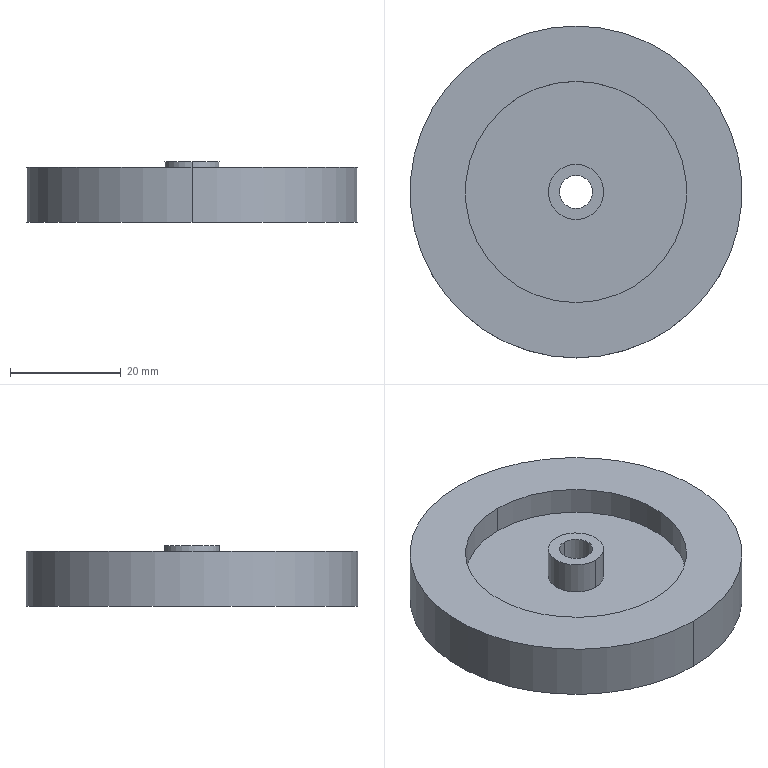Component | SolidWorks | DriveStripPlate-1 | 1 solid | 12 faces | box 60 x 60 x 11 mm | volume 22151 mm3 | cylinder 8 | plane 4 | commonest cylinder face diameters 10 x2 6 x2 60 x2 40 x2
build123d program:
from build123d import *

# Parameters (mm, degrees)
SKETCH1_R           = 30
SKETCH1_R_2         = 20
BOSS_EXTRUDE1_DEPTH = 10
SKETCH2_R           = 20
SKETCH2_R_2         = 3
BOSS_EXTRUDE2_DEPTH = 5
SKETCH3_R           = 5
SKETCH3_R_2         = 3
BOSS_EXTRUDE3_DEPTH = 6


with BuildPart() as part:
    # Sketch1 → Boss-Extrude1 (new body)
    with BuildSketch(Plane.XY):
        with Locations((71.434, 305)):
            Circle(SKETCH1_R)
        with Locations((71.434, 305)):
            Circle(SKETCH1_R_2, mode=Mode.SUBTRACT)
    extrude(amount=BOSS_EXTRUDE1_DEPTH)

    # Sketch2 → Boss-Extrude2 (add)
    with BuildSketch(Plane(origin=(0, 0, 0), x_dir=(-1, 0, 0), z_dir=(0, 0, -1))):
        with Locations((-71.434, 305)):
            Circle(SKETCH2_R)
        with Locations((-71.434, 305)):
            Circle(SKETCH2_R_2, mode=Mode.SUBTRACT)
    extrude(amount=-BOSS_EXTRUDE2_DEPTH)

    # Sketch3 → Boss-Extrude3 (add)
    with BuildSketch(Plane.XY.offset(5)):
        with Locations(Location((71.434, 305, 0), (0, 0, 180))):
            Circle(SKETCH3_R)
        with Locations(Location((71.434, 305, 0), (0, 0, 180))):
            Circle(SKETCH3_R_2, mode=Mode.SUBTRACT)
    extrude(amount=BOSS_EXTRUDE3_DEPTH)


solid = part.part

# Placed as in the assembly
solid = solid.moved(Location((-511.434, -213, 50), (0, 0, 0)))
STEP:
#1=CARTESIAN_POINT('',(-17.323,3.819,2.402));
#2=VERTEX_POINT('',#1);
#3=CARTESIAN_POINT('',(-17.323,3.425,2.402));
#4=VERTEX_POINT('',#3);
#5=CARTESIAN_POINT('',(-17.323,3.622,2.402));
#6=DIRECTION('',(0.,0.,1.));
#7=DIRECTION('',(0.,1.,0.));
#8=AXIS2_PLACEMENT_3D('',#5,#6,#7);
#9=CIRCLE('',#8,0.1969);
#10=EDGE_CURVE('',#2,#4,#9,.T.);
#11=ORIENTED_EDGE('',*,*,#10,.F.);
#12=CARTESIAN_POINT('',(-17.323,3.819,2.165));
#13=VERTEX_POINT('',#12);
#14=CARTESIAN_POINT('',(-17.323,3.819,2.402));
#15=DIRECTION('',(0.,0.,-1.));
#16=VECTOR('',#15,39.37);
#17=LINE('',#14,#16);
#18=EDGE_CURVE('',#2,#13,#17,.T.);
#19=ORIENTED_EDGE('',*,*,#18,.T.);
#20=CARTESIAN_POINT('',(-17.323,3.425,2.165));
#21=VERTEX_POINT('',#20);
#22=CARTESIAN_POINT('',(-17.323,3.622,2.165));
#23=DIRECTION('',(0.,0.,1.));
#24=DIRECTION('',(0.,-1.,0.));
#25=AXIS2_PLACEMENT_3D('',#22,#23,#24);
#26=CIRCLE('',#25,0.1969);
#27=EDGE_CURVE('',#13,#21,#26,.T.);
#28=ORIENTED_EDGE('',*,*,#27,.T.);
#29=CARTESIAN_POINT('',(-17.323,3.425,2.402));
#30=DIRECTION('',(0.,0.,-1.));
#31=VECTOR('',#30,39.37);
#32=LINE('',#29,#31);
#33=EDGE_CURVE('',#4,#21,#32,.T.);
#34=ORIENTED_EDGE('',*,*,#33,.F.);
#35=EDGE_LOOP('',(#11,#19,#28,#34));
#36=FACE_OUTER_BOUND('',#35,.T.);
#37=CARTESIAN_POINT('',(-17.323,3.622,2.402));
#38=DIRECTION('',(0.,0.,-1.));
#39=DIRECTION('',(0.,-1.,0.));
#40=AXIS2_PLACEMENT_3D('',#37,#38,#39);
#41=CYLINDRICAL_SURFACE('',#40,0.1969);
#42=ADVANCED_FACE('',(#36),#41,.T.);
#43=CARTESIAN_POINT('',(-17.323,3.504,2.402));
#44=VERTEX_POINT('',#43);
#45=CARTESIAN_POINT('',(-17.323,3.74,2.402));
#46=VERTEX_POINT('',#45);
#47=CARTESIAN_POINT('',(-17.323,3.622,2.402));
#48=DIRECTION('',(0.,0.,1.));
#49=DIRECTION('',(0.,1.,0.));
#50=AXIS2_PLACEMENT_3D('',#47,#48,#49);
#51=CIRCLE('',#50,0.1181);
#52=EDGE_CURVE('',#44,#46,#51,.T.);
#53=ORIENTED_EDGE('',*,*,#52,.T.);
#54=CARTESIAN_POINT('',(-17.323,3.74,1.969));
#55=VERTEX_POINT('',#54);
#56=CARTESIAN_POINT('',(-17.323,3.74,2.165));
#57=DIRECTION('',(0.,0.,-1.));
#58=VECTOR('',#57,39.37);
#59=LINE('',#56,#58);
#60=EDGE_CURVE('',#46,#55,#59,.T.);
#61=ORIENTED_EDGE('',*,*,#60,.T.);
#62=CARTESIAN_POINT('',(-17.323,3.504,1.969));
#63=VERTEX_POINT('',#62);
#64=CARTESIAN_POINT('',(-17.323,3.622,1.969));
#65=DIRECTION('',(0.,0.,-1.));
#66=DIRECTION('',(0.,-1.,0.));
#67=AXIS2_PLACEMENT_3D('',#64,#65,#66);
#68=CIRCLE('',#67,0.1181);
#69=EDGE_CURVE('',#55,#63,#68,.T.);
#70=ORIENTED_EDGE('',*,*,#69,.T.);
#71=CARTESIAN_POINT('',(-17.323,3.504,2.165));
#72=DIRECTION('',(0.,0.,-1.));
#73=VECTOR('',#72,39.37);
#74=LINE('',#71,#73);
#75=EDGE_CURVE('',#44,#63,#74,.T.);
#76=ORIENTED_EDGE('',*,*,#75,.F.);
#77=EDGE_LOOP('',(#53,#61,#70,#76));
#78=FACE_OUTER_BOUND('',#77,.T.);
#79=CARTESIAN_POINT('',(-17.323,3.622,2.165));
#80=DIRECTION('',(0.,0.,-1.));
#81=DIRECTION('',(0.,-1.,0.));
#82=AXIS2_PLACEMENT_3D('',#79,#80,#81);
#83=CYLINDRICAL_SURFACE('',#82,0.1181);
#84=ADVANCED_FACE('',(#78),#83,.F.);
#85=CARTESIAN_POINT('',(-17.323,4.803,2.362));
#86=VERTEX_POINT('',#85);
#87=CARTESIAN_POINT('',(-17.323,2.441,2.362));
#88=VERTEX_POINT('',#87);
#89=CARTESIAN_POINT('',(-17.323,3.622,2.362));
#90=DIRECTION('',(0.,0.,1.));
#91=DIRECTION('',(0.,1.,0.));
#92=AXIS2_PLACEMENT_3D('',#89,#90,#91);
#93=CIRCLE('',#92,1.181);
#94=EDGE_CURVE('',#86,#88,#93,.T.);
#95=ORIENTED_EDGE('',*,*,#94,.F.);
#96=CARTESIAN_POINT('',(-17.323,4.803,1.969));
#97=VERTEX_POINT('',#96);
#98=CARTESIAN_POINT('',(-17.323,4.803,2.362));
#99=DIRECTION('',(0.,0.,-1.));
#100=VECTOR('',#99,39.37);
#101=LINE('',#98,#100);
#102=EDGE_CURVE('',#86,#97,#101,.T.);
#103=ORIENTED_EDGE('',*,*,#102,.T.);
#104=CARTESIAN_POINT('',(-17.323,2.441,1.969));
#105=VERTEX_POINT('',#104);
#106=CARTESIAN_POINT('',(-17.323,3.622,1.969));
#107=DIRECTION('',(0.,0.,1.));
#108=DIRECTION('',(0.,1.,0.));
#109=AXIS2_PLACEMENT_3D('',#106,#107,#108);
#110=CIRCLE('',#109,1.181);
#111=EDGE_CURVE('',#97,#105,#110,.T.);
#112=ORIENTED_EDGE('',*,*,#111,.T.);
#113=CARTESIAN_POINT('',(-17.323,2.441,2.362));
#114=DIRECTION('',(0.,0.,-1.));
#115=VECTOR('',#114,39.37);
#116=LINE('',#113,#115);
#117=EDGE_CURVE('',#88,#105,#116,.T.);
#118=ORIENTED_EDGE('',*,*,#117,.F.);
#119=EDGE_LOOP('',(#95,#103,#112,#118));
#120=FACE_OUTER_BOUND('',#119,.T.);
#121=CARTESIAN_POINT('',(-17.323,3.622,2.362));
#122=DIRECTION('',(0.,0.,-1.));
#123=DIRECTION('',(0.,-1.,0.));
#124=AXIS2_PLACEMENT_3D('',#121,#122,#123);
#125=CYLINDRICAL_SURFACE('',#124,1.181);
#126=ADVANCED_FACE('',(#120),#125,.T.);
#127=CARTESIAN_POINT('',(-17.323,2.835,2.362));
#128=VERTEX_POINT('',#127);
#129=CARTESIAN_POINT('',(-17.323,4.409,2.362));
#130=VERTEX_POINT('',#129);
#131=CARTESIAN_POINT('',(-17.323,3.622,2.362));
#132=DIRECTION('',(0.,0.,1.));
#133=DIRECTION('',(0.,1.,0.));
#134=AXIS2_PLACEMENT_3D('',#131,#132,#133);
#135=CIRCLE('',#134,0.7874);
#136=EDGE_CURVE('',#128,#130,#135,.T.);
#137=ORIENTED_EDGE('',*,*,#136,.T.);
#138=CARTESIAN_POINT('',(-17.323,4.409,2.165));
#139=VERTEX_POINT('',#138);
#140=CARTESIAN_POINT('',(-17.323,4.409,2.362));
#141=DIRECTION('',(0.,0.,-1.));
#142=VECTOR('',#141,39.37);
#143=LINE('',#140,#142);
#144=EDGE_CURVE('',#130,#139,#143,.T.);
#145=ORIENTED_EDGE('',*,*,#144,.T.);
#146=CARTESIAN_POINT('',(-17.323,2.835,2.165));
#147=VERTEX_POINT('',#146);
#148=CARTESIAN_POINT('',(-17.323,3.622,2.165));
#149=DIRECTION('',(0.,0.,-1.));
#150=DIRECTION('',(0.,-1.,0.));
#151=AXIS2_PLACEMENT_3D('',#148,#149,#150);
#152=CIRCLE('',#151,0.7874);
#153=EDGE_CURVE('',#139,#147,#152,.T.);
#154=ORIENTED_EDGE('',*,*,#153,.T.);
#155=CARTESIAN_POINT('',(-17.323,2.835,2.362));
#156=DIRECTION('',(0.,0.,-1.));
#157=VECTOR('',#156,39.37);
#158=LINE('',#155,#157);
#159=EDGE_CURVE('',#128,#147,#158,.T.);
#160=ORIENTED_EDGE('',*,*,#159,.F.);
#161=EDGE_LOOP('',(#137,#145,#154,#160));
#162=FACE_OUTER_BOUND('',#161,.T.);
#163=CARTESIAN_POINT('',(-17.323,3.622,2.362));
#164=DIRECTION('',(0.,0.,-1.));
#165=DIRECTION('',(0.,-1.,0.));
#166=AXIS2_PLACEMENT_3D('',#163,#164,#165);
#167=CYLINDRICAL_SURFACE('',#166,0.7874);
#168=ADVANCED_FACE('',(#162),#167,.F.);
#169=CARTESIAN_POINT('',(-17.323,3.622,2.165));
#170=DIRECTION('',(0.,0.,-1.));
#171=DIRECTION('',(0.,-1.,0.));
#172=AXIS2_PLACEMENT_3D('',#169,#170,#171);
#173=CIRCLE('',#172,0.7874);
#174=EDGE_CURVE('',#147,#139,#173,.T.);
#175=ORIENTED_EDGE('',*,*,#174,.F.);
#176=ORIENTED_EDGE('',*,*,#153,.F.);
#177=EDGE_LOOP('',(#175,#176));
#178=FACE_OUTER_BOUND('',#177,.T.);
#179=CARTESIAN_POINT('',(-17.323,3.622,2.165));
#180=DIRECTION('',(0.,0.,1.));
#181=DIRECTION('',(0.,-1.,0.));
#182=AXIS2_PLACEMENT_3D('',#179,#180,#181);
#183=CIRCLE('',#182,0.1969);
#184=EDGE_CURVE('',#21,#13,#183,.T.);
#185=ORIENTED_EDGE('',*,*,#184,.F.);
#186=ORIENTED_EDGE('',*,*,#27,.F.);
#187=EDGE_LOOP('',(#185,#186));
#188=FACE_BOUND('',#187,.T.);
#189=CARTESIAN_POINT('',(-17.323,3.622,2.165));
#190=DIRECTION('',(0.,0.,-1.));
#191=DIRECTION('',(0.,-1.,0.));
#192=AXIS2_PLACEMENT_3D('',#189,#190,#191);
#193=PLANE('',#192);
#194=ADVANCED_FACE('',(#178,#188),#193,.F.);
#195=ORIENTED_EDGE('',*,*,#144,.F.);
#196=CARTESIAN_POINT('',(-17.323,3.622,2.362));
#197=DIRECTION('',(0.,0.,1.));
#198=DIRECTION('',(0.,1.,0.));
#199=AXIS2_PLACEMENT_3D('',#196,#197,#198);
#200=CIRCLE('',#199,0.7874);
#201=EDGE_CURVE('',#130,#128,#200,.T.);
#202=ORIENTED_EDGE('',*,*,#201,.T.);
#203=ORIENTED_EDGE('',*,*,#159,.T.);
#204=ORIENTED_EDGE('',*,*,#174,.T.);
#205=EDGE_LOOP('',(#195,#202,#203,#204));
#206=FACE_OUTER_BOUND('',#205,.T.);
#207=CARTESIAN_POINT('',(-17.323,3.622,2.362));
#208=DIRECTION('',(0.,0.,-1.));
#209=DIRECTION('',(0.,-1.,0.));
#210=AXIS2_PLACEMENT_3D('',#207,#208,#209);
#211=CYLINDRICAL_SURFACE('',#210,0.7874);
#212=ADVANCED_FACE('',(#206),#211,.F.);
#213=CARTESIAN_POINT('',(-17.323,3.622,2.362));
#214=DIRECTION('',(0.,0.,1.));
#215=DIRECTION('',(0.,1.,0.));
#216=AXIS2_PLACEMENT_3D('',#213,#214,#215);
#217=CIRCLE('',#216,1.181);
#218=EDGE_CURVE('',#88,#86,#217,.T.);
#219=ORIENTED_EDGE('',*,*,#218,.T.);
#220=ORIENTED_EDGE('',*,*,#94,.T.);
#221=EDGE_LOOP('',(#219,#220));
#222=FACE_OUTER_BOUND('',#221,.T.);
#223=ORIENTED_EDGE('',*,*,#136,.F.);
#224=ORIENTED_EDGE('',*,*,#201,.F.);
#225=EDGE_LOOP('',(#223,#224));
#226=FACE_BOUND('',#225,.T.);
#227=CARTESIAN_POINT('',(-17.323,3.622,2.362));
#228=DIRECTION('',(0.,0.,1.));
#229=DIRECTION('',(0.,1.,0.));
#230=AXIS2_PLACEMENT_3D('',#227,#228,#229);
#231=PLANE('',#230);
#232=ADVANCED_FACE('',(#222,#226),#231,.T.);
#233=CARTESIAN_POINT('',(-17.323,3.622,1.969));
#234=DIRECTION('',(0.,0.,1.));
#235=DIRECTION('',(0.,1.,0.));
#236=AXIS2_PLACEMENT_3D('',#233,#234,#235);
#237=CIRCLE('',#236,1.181);
#238=EDGE_CURVE('',#105,#97,#237,.T.);
#239=ORIENTED_EDGE('',*,*,#238,.F.);
#240=ORIENTED_EDGE('',*,*,#111,.F.);
#241=EDGE_LOOP('',(#239,#240));
#242=FACE_OUTER_BOUND('',#241,.T.);
#243=CARTESIAN_POINT('',(-17.323,3.622,1.969));
#244=DIRECTION('',(0.,0.,-1.));
#245=DIRECTION('',(0.,-1.,0.));
#246=AXIS2_PLACEMENT_3D('',#243,#244,#245);
#247=CIRCLE('',#246,0.1181);
#248=EDGE_CURVE('',#63,#55,#247,.T.);
#249=ORIENTED_EDGE('',*,*,#248,.F.);
#250=ORIENTED_EDGE('',*,*,#69,.F.);
#251=EDGE_LOOP('',(#249,#250));
#252=FACE_BOUND('',#251,.T.);
#253=CARTESIAN_POINT('',(-17.323,3.622,1.969));
#254=DIRECTION('',(0.,0.,1.));
#255=DIRECTION('',(0.,1.,0.));
#256=AXIS2_PLACEMENT_3D('',#253,#254,#255);
#257=PLANE('',#256);
#258=ADVANCED_FACE('',(#242,#252),#257,.F.);
#259=ORIENTED_EDGE('',*,*,#102,.F.);
#260=ORIENTED_EDGE('',*,*,#218,.F.);
#261=ORIENTED_EDGE('',*,*,#117,.T.);
#262=ORIENTED_EDGE('',*,*,#238,.T.);
#263=EDGE_LOOP('',(#259,#260,#261,#262));
#264=FACE_OUTER_BOUND('',#263,.T.);
#265=CARTESIAN_POINT('',(-17.323,3.622,2.362));
#266=DIRECTION('',(0.,0.,-1.));
#267=DIRECTION('',(0.,-1.,0.));
#268=AXIS2_PLACEMENT_3D('',#265,#266,#267);
#269=CYLINDRICAL_SURFACE('',#268,1.181);
#270=ADVANCED_FACE('',(#264),#269,.T.);
#271=ORIENTED_EDGE('',*,*,#60,.F.);
#272=CARTESIAN_POINT('',(-17.323,3.622,2.402));
#273=DIRECTION('',(0.,0.,1.));
#274=DIRECTION('',(0.,1.,0.));
#275=AXIS2_PLACEMENT_3D('',#272,#273,#274);
#276=CIRCLE('',#275,0.1181);
#277=EDGE_CURVE('',#46,#44,#276,.T.);
#278=ORIENTED_EDGE('',*,*,#277,.T.);
#279=ORIENTED_EDGE('',*,*,#75,.T.);
#280=ORIENTED_EDGE('',*,*,#248,.T.);
#281=EDGE_LOOP('',(#271,#278,#279,#280));
#282=FACE_OUTER_BOUND('',#281,.T.);
#283=CARTESIAN_POINT('',(-17.323,3.622,2.165));
#284=DIRECTION('',(0.,0.,-1.));
#285=DIRECTION('',(0.,-1.,0.));
#286=AXIS2_PLACEMENT_3D('',#283,#284,#285);
#287=CYLINDRICAL_SURFACE('',#286,0.1181);
#288=ADVANCED_FACE('',(#282),#287,.F.);
#289=CARTESIAN_POINT('',(-17.323,3.622,2.402));
#290=DIRECTION('',(0.,0.,1.));
#291=DIRECTION('',(0.,1.,0.));
#292=AXIS2_PLACEMENT_3D('',#289,#290,#291);
#293=CIRCLE('',#292,0.1969);
#294=EDGE_CURVE('',#4,#2,#293,.T.);
#295=ORIENTED_EDGE('',*,*,#294,.T.);
#296=ORIENTED_EDGE('',*,*,#10,.T.);
#297=EDGE_LOOP('',(#295,#296));
#298=FACE_OUTER_BOUND('',#297,.T.);
#299=ORIENTED_EDGE('',*,*,#52,.F.);
#300=ORIENTED_EDGE('',*,*,#277,.F.);
#301=EDGE_LOOP('',(#299,#300));
#302=FACE_BOUND('',#301,.T.);
#303=CARTESIAN_POINT('',(-17.323,3.622,2.402));
#304=DIRECTION('',(0.,0.,1.));
#305=DIRECTION('',(0.,1.,0.));
#306=AXIS2_PLACEMENT_3D('',#303,#304,#305);
#307=PLANE('',#306);
#308=ADVANCED_FACE('',(#298,#302),#307,.T.);
#309=ORIENTED_EDGE('',*,*,#18,.F.);
#310=ORIENTED_EDGE('',*,*,#294,.F.);
#311=ORIENTED_EDGE('',*,*,#33,.T.);
#312=ORIENTED_EDGE('',*,*,#184,.T.);
#313=EDGE_LOOP('',(#309,#310,#311,#312));
#314=FACE_OUTER_BOUND('',#313,.T.);
#315=CARTESIAN_POINT('',(-17.323,3.622,2.402));
#316=DIRECTION('',(0.,0.,-1.));
#317=DIRECTION('',(0.,-1.,0.));
#318=AXIS2_PLACEMENT_3D('',#315,#316,#317);
#319=CYLINDRICAL_SURFACE('',#318,0.1969);
#320=ADVANCED_FACE('',(#314),#319,.T.);
#321=CLOSED_SHELL('',(#42,#84,#126,#168,#194,#212,#232,#258,#270,#288,#308,#320));
#322=MANIFOLD_SOLID_BREP('',#321);
#323=CARTESIAN_POINT('',(0.,0.,0.));
#324=DIRECTION('',(0.,0.,1.));
#325=DIRECTION('',(1.,0.,0.));
#326=AXIS2_PLACEMENT_3D('',#323,#324,#325);
#327=(LENGTH_UNIT()NAMED_UNIT(*)SI_UNIT($,.METRE.));
#328=LENGTH_MEASURE_WITH_UNIT(LENGTH_MEASURE(0.0254),#327);
#329=DIMENSIONAL_EXPONENTS(1.,0.,0.,0.,0.,0.,0.);
#330=(CONVERSION_BASED_UNIT('',#328)LENGTH_UNIT()NAMED_UNIT(#329));
#331=UNCERTAINTY_MEASURE_WITH_UNIT(LENGTH_MEASURE(0.00001),#330,'','');
#332=(NAMED_UNIT(*)PLANE_ANGLE_UNIT()SI_UNIT($,.RADIAN.));
#333=(NAMED_UNIT(*)SI_UNIT($,.STERADIAN.)SOLID_ANGLE_UNIT());
#334=(GEOMETRIC_REPRESENTATION_CONTEXT(3)GLOBAL_UNCERTAINTY_ASSIGNED_CONTEXT((#331))GLOBAL_UNIT_ASSIGNED_CONTEXT((#330,#332,#333))REPRESENTATION_CONTEXT('',''));
#335=ADVANCED_BREP_SHAPE_REPRESENTATION('',(#322,#326),#334);
#336=COLOUR_RGB('',0.7922,0.8196,0.9333);
#337=FILL_AREA_STYLE_COLOUR('',#336);
#338=FILL_AREA_STYLE('',(#337));
#339=SURFACE_STYLE_FILL_AREA(#338);
#340=SURFACE_SIDE_STYLE('',(#339));
#341=SURFACE_STYLE_USAGE(.BOTH.,#340);
#342=PRESENTATION_STYLE_ASSIGNMENT((#341));
#343=STYLED_ITEM('',(#342),#322);
#344=PRESENTATION_LAYER_ASSIGNMENT('','',(#343));
#345=(LENGTH_UNIT()NAMED_UNIT(*)SI_UNIT($,.METRE.));
#346=LENGTH_MEASURE_WITH_UNIT(LENGTH_MEASURE(0.0254),#345);
#347=DIMENSIONAL_EXPONENTS(1.,0.,0.,0.,0.,0.,0.);
#348=(CONVERSION_BASED_UNIT('',#346)LENGTH_UNIT()NAMED_UNIT(#347));
#349=UNCERTAINTY_MEASURE_WITH_UNIT(LENGTH_MEASURE(0.00001),#348,'','');
#350=(NAMED_UNIT(*)PLANE_ANGLE_UNIT()SI_UNIT($,.RADIAN.));
#351=(NAMED_UNIT(*)SI_UNIT($,.STERADIAN.)SOLID_ANGLE_UNIT());
#352=(GEOMETRIC_REPRESENTATION_CONTEXT(3)GLOBAL_UNCERTAINTY_ASSIGNED_CONTEXT((#349))GLOBAL_UNIT_ASSIGNED_CONTEXT((#348,#350,#351))REPRESENTATION_CONTEXT('',''));
#353=MECHANICAL_DESIGN_GEOMETRIC_PRESENTATION_REPRESENTATION('',(#343),#352);